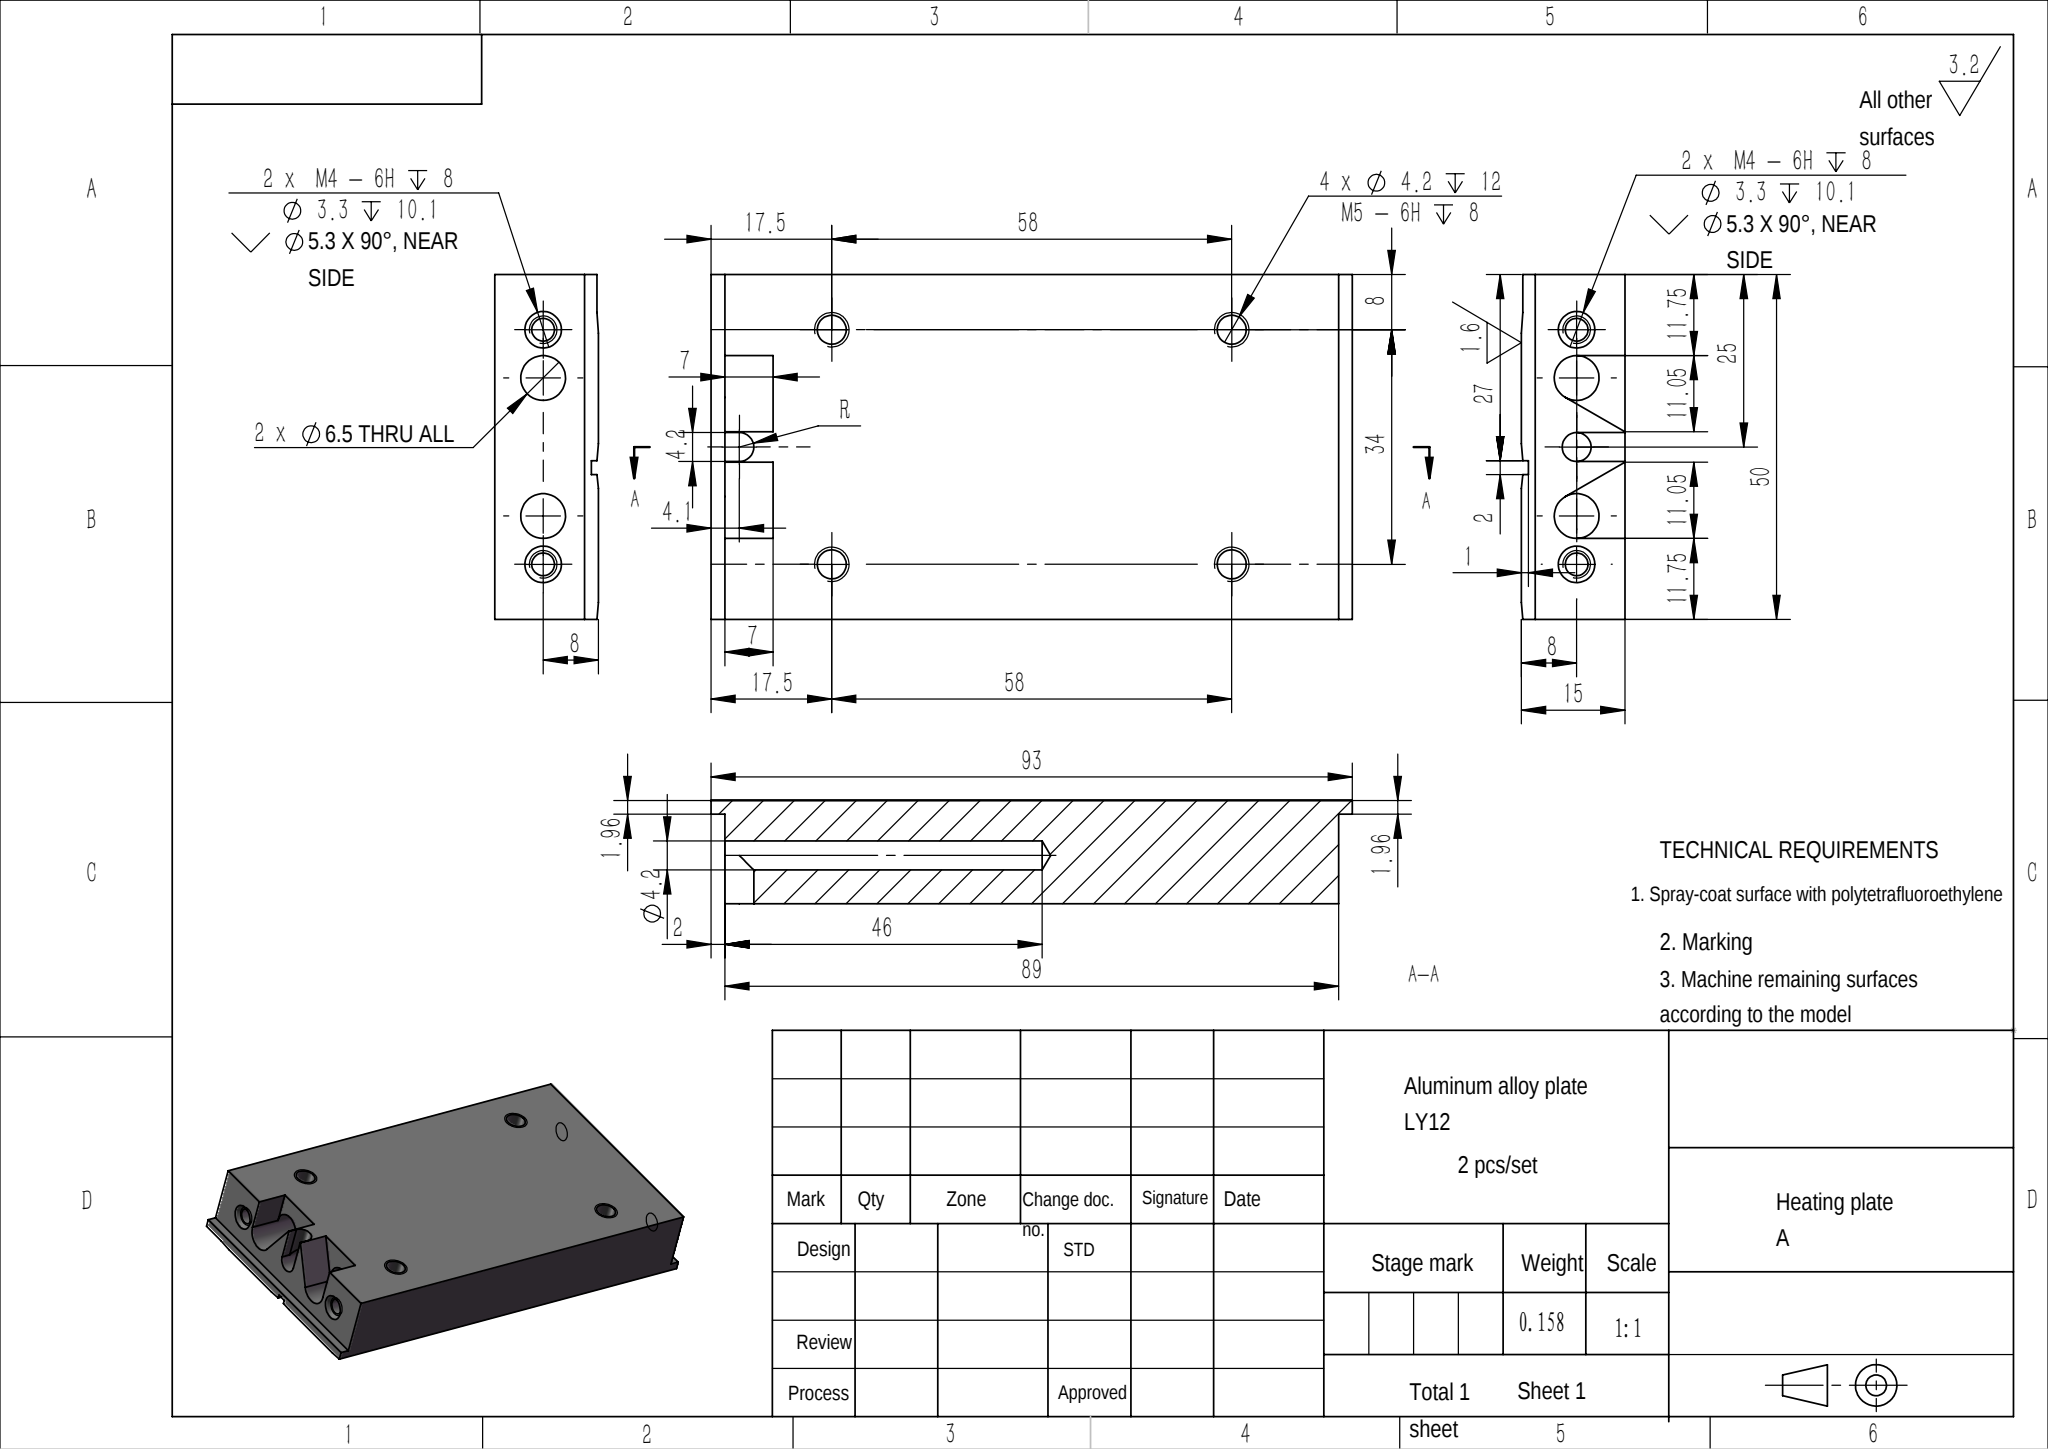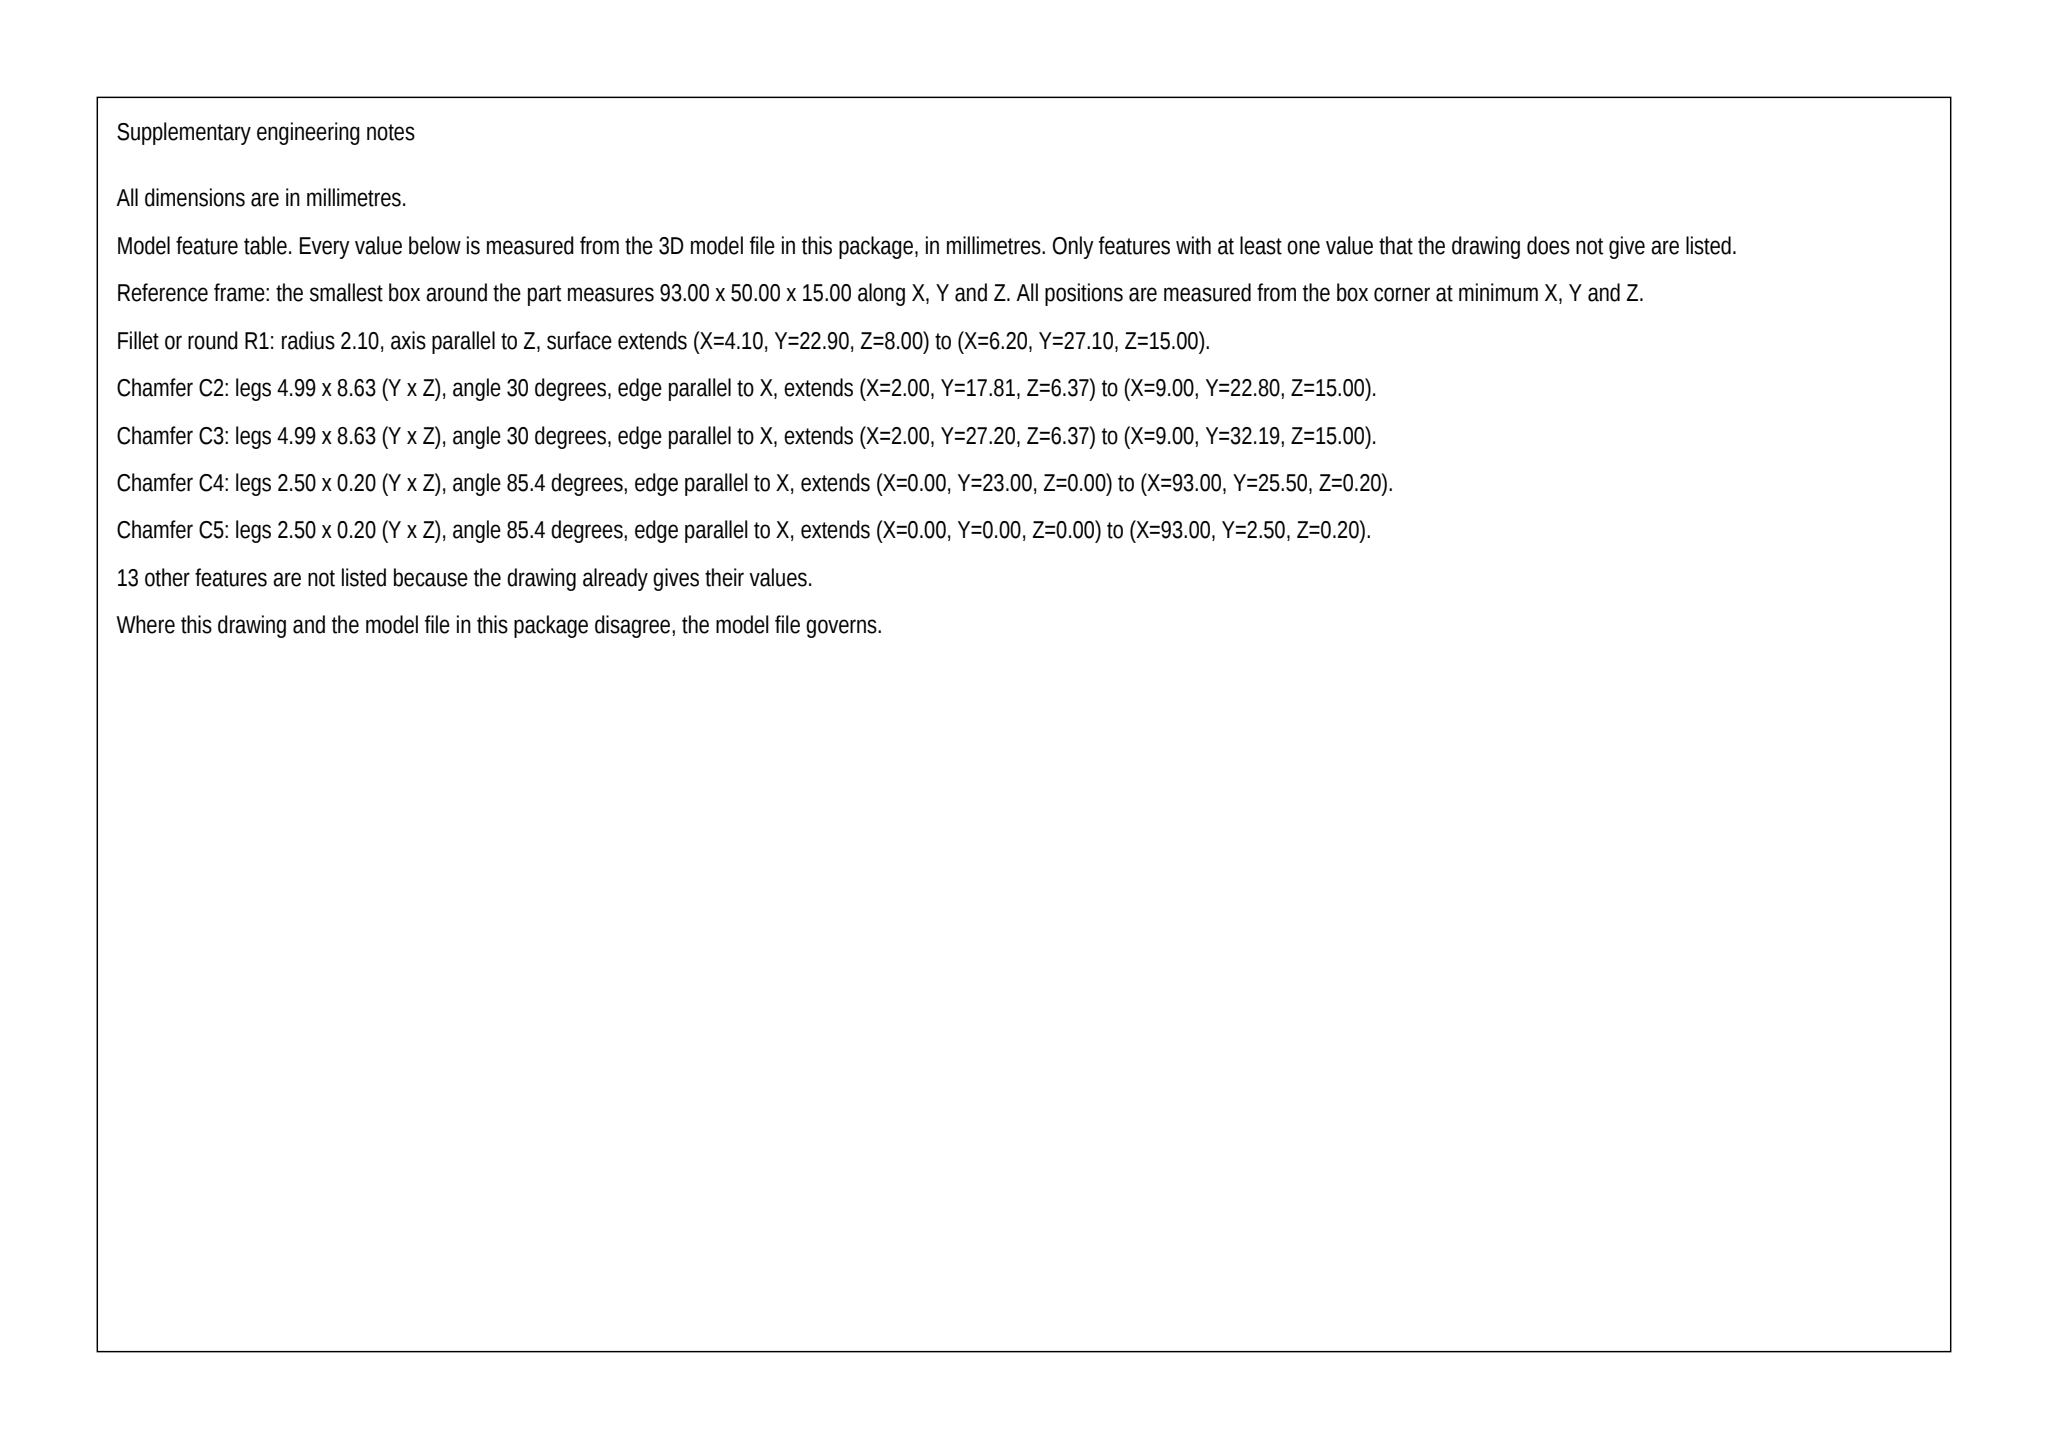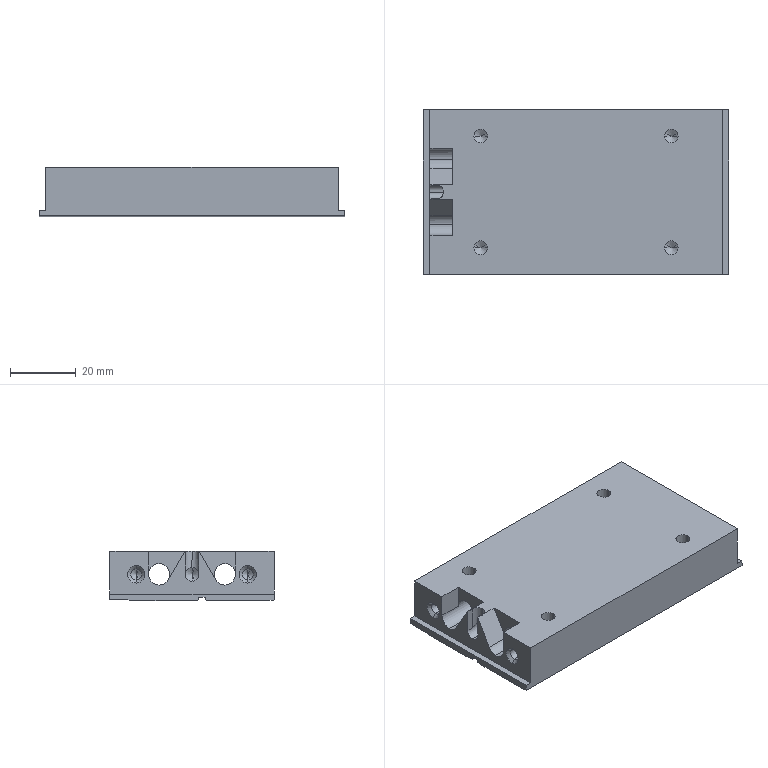Part | SolidWorks | mm | material Aluminum alloy plate LY12 | 1 solid | 77 faces | box 93 x 50 x 15 mm | volume 58409 mm3 | plane 27 | cone 26 | cylinder 24 | commonest cylinder face diameters 4.2 x12 3.3 x8 6.5 x4
build123d program:
from build123d import *

# Parameters (mm, degrees)
SKETCH1_W                      = 93
SKETCH1_H                      = 50
BOSS_EXTRUDE1_DEPTH            = 15
SKETCH2_W                      = 13.775
SKETCH2_H                      = 59.635
SKETCH2_W_2                    = 21.67
SKETCH2_H_2                    = 65.682
CUT_EXTRUDE1_DEPTH             = 13
F_6_5_6_5_DIAMETER_HOLE1_D     = 6.5
M4_TAPPED_HOLE1_D              = 3.3
M4_TAPPED_HOLE1_DEPTH          = 10.1
M4_TAPPED_HOLE1_CSINK_D        = 5.3
M4_TAPPED_HOLE1_CSINK_ANGLE    = 90
M4_TAPPED_HOLE1_TIP            = 0.9914
F_4_2_4_2_DIAMETER_HOLE1_D     = 4.2
F_4_2_4_2_DIAMETER_HOLE1_DEPTH = 46
F_4_2_4_2_DIAMETER_HOLE1_TIP   = 1.262
M4_TAPPED_HOLE2_D              = 3.3
M4_TAPPED_HOLE2_DEPTH          = 10.1
M4_TAPPED_HOLE2_CSINK_D        = 5.3
M4_TAPPED_HOLE2_CSINK_ANGLE    = 90
M4_TAPPED_HOLE2_TIP            = 0.9914
CUT_EXTRUDE3_REACH             = 56.884
CUT_EXTRUDE3_END_RADIUS        = 2.1
CUT_EXTRUDE4_START             = -7
CUT_EXTRUDE4_DEPTH             = 7
SKETCH17_W                     = 5.449
SKETCH17_H                     = 2
CUT_EXTRUDE5_DEPTH             = 98.463
M5_TAPPED_HOLE1_D              = 4.2
M5_TAPPED_HOLE1_DEPTH          = 12
M5_TAPPED_HOLE1_TIP            = 1.262
CUT_EXTRUDE6_DEPTH             = 98.463


with BuildPart() as part:
    # Sketch1 → Boss-Extrude1 (new body)
    with BuildSketch(Plane.XY):
        Rectangle(SKETCH1_W, SKETCH1_H)
    extrude(amount=-BOSS_EXTRUDE1_DEPTH)

    # Sketch2 → Cut-Extrude1 (cut)
    with BuildSketch(Plane.XY):
        with Locations((-51.387, 0.6719)):
            Rectangle(SKETCH2_W, SKETCH2_H)
        with Locations((55.335, -0.504)):
            Rectangle(SKETCH2_W_2, SKETCH2_H_2)
    extrude(amount=-CUT_EXTRUDE1_DEPTH, mode=Mode.SUBTRACT)

    # 6.5 _6.5_ Diameter Hole1 (through all)
    with Locations(Plane.ZY.offset(44.5)):
        with Locations((-7, 10), (-7, -10)):
            Hole(F_6_5_6_5_DIAMETER_HOLE1_D / 2)

    # M4 Tapped Hole1
    with Locations(Plane.ZY.offset(44.5)):
        with Locations((-7, 17), (-7, -17)):
            CounterSinkHole(M4_TAPPED_HOLE1_D / 2, M4_TAPPED_HOLE1_CSINK_D / 2, depth=M4_TAPPED_HOLE1_DEPTH, counter_sink_angle=M4_TAPPED_HOLE1_CSINK_ANGLE)
            with Locations((0, 0, -(M4_TAPPED_HOLE1_DEPTH + M4_TAPPED_HOLE1_TIP / 2))):  # 118° drill point
                Cone(0, M4_TAPPED_HOLE1_D / 2, M4_TAPPED_HOLE1_TIP, mode=Mode.SUBTRACT)

    # 4.2 _4.2_ Diameter Hole1
    with Locations(Plane.ZY.offset(44.5)):
        with Locations((-7, 0)):
            Hole(F_4_2_4_2_DIAMETER_HOLE1_D / 2, depth=F_4_2_4_2_DIAMETER_HOLE1_DEPTH)
            with Locations((0, 0, -(F_4_2_4_2_DIAMETER_HOLE1_DEPTH + F_4_2_4_2_DIAMETER_HOLE1_TIP / 2))):  # 118° drill point
                Cone(0, F_4_2_4_2_DIAMETER_HOLE1_D / 2, F_4_2_4_2_DIAMETER_HOLE1_TIP, mode=Mode.SUBTRACT)

    # M4 Tapped Hole2
    with Locations(Plane(origin=(44.5, 0, 0), x_dir=(0, 0, -1), z_dir=(1, 0, 0))):
        with Locations((7, 17), (7, -17)):
            CounterSinkHole(M4_TAPPED_HOLE2_D / 2, M4_TAPPED_HOLE2_CSINK_D / 2, depth=M4_TAPPED_HOLE2_DEPTH, counter_sink_angle=M4_TAPPED_HOLE2_CSINK_ANGLE)
            with Locations((0, 0, -(M4_TAPPED_HOLE2_DEPTH + M4_TAPPED_HOLE2_TIP / 2))):  # 118° drill point
                Cone(0, M4_TAPPED_HOLE2_D / 2, M4_TAPPED_HOLE2_TIP, mode=Mode.SUBTRACT)

    # Cut-Extrude3: up to this cylinder (the profile starts outside it)
    cut_extrude3_end = Plane(origin=(-42.596, 0, -7), z_dir=(-1, 0, 0)) * Cylinder(CUT_EXTRUDE3_END_RADIUS, 118.968, mode=Mode.PRIVATE)
    # Sketch15 → Cut-Extrude3 (cut, up to the surface)
    with BuildSketch(Plane.XY, mode=Mode.PRIVATE) as cut_extrude3_sk1:
        with BuildLine():
            Line((-42.4, 2.1), (-44.5, 2.1))
            Line((-44.5, 2.1), (-44.5, -2.1))
            Line((-44.5, -2.1), (-42.4, -2.1))
            ThreePointArc((-42.4, -2.1), (-40.3, 0), (-42.4, 2.1))
        make_face()
    cut_extrude3_tool1 = extrude(cut_extrude3_sk1.sketch, amount=-CUT_EXTRUDE3_REACH, mode=Mode.PRIVATE) - cut_extrude3_end
    add(cut_extrude3_tool1.solids().sort_by_distance((-42.596, 0, 0))[0], mode=Mode.SUBTRACT)

    # Sketch16 → Cut-Extrude4 (cut)
    with BuildSketch(Plane.ZY.offset(44.5).offset(CUT_EXTRUDE4_START)):
        with BuildLine():
            Line((0, -13.25), (0, -2.2))
            Line((0, -2.2), (-8.626, -7.186))
            ThreePointArc((-8.626, -7.186), (-10.139, -10.842), (-7, -13.25))
            Line((-7, -13.25), (0, -13.25))
        make_face()
        with BuildLine():
            Line((0, 13.25), (0, 2.2))
            Line((0, 2.2), (-8.626, 7.186))
            ThreePointArc((-8.626, 7.186), (-10.139, 10.842), (-7, 13.25))
            Line((-7, 13.25), (0, 13.25))
        make_face()
    extrude(amount=CUT_EXTRUDE4_DEPTH, mode=Mode.SUBTRACT)

    # Sketch17 → Cut-Extrude5 (cut, through all)
    with BuildSketch(Plane.ZY.offset(46.5)):
        with Locations((-16.724, -3)):
            Rectangle(SKETCH17_W, SKETCH17_H)
    extrude(amount=-CUT_EXTRUDE5_DEPTH, mode=Mode.SUBTRACT)

    # M5 Tapped Hole1
    with Locations(Plane.XY):
        with Locations((-29, 17), (29, 17), (-29, -17), (29, -17)):
            Hole(M5_TAPPED_HOLE1_D / 2, depth=M5_TAPPED_HOLE1_DEPTH)
            with Locations((0, 0, -(M5_TAPPED_HOLE1_DEPTH + M5_TAPPED_HOLE1_TIP / 2))):  # 118° drill point
                Cone(0, M5_TAPPED_HOLE1_D / 2, M5_TAPPED_HOLE1_TIP, mode=Mode.SUBTRACT)

    # Sketch20 → Cut-Extrude6 (cut, through all)
    with BuildSketch(Plane(origin=(46.5, 0, 0), x_dir=(0, 0, -1), z_dir=(1, 0, 0))):
        Polygon((14.8, 25), (14.8, 19.5), (15, 16.5), (15, 25), align=None)
        Polygon((15, 0.5), (14.8, -2), (15, -2), align=None)
        Polygon((14.8, -4), (15, -6), (15, -4), align=None)
        Polygon((15, -22.5), (14.8, -25), (15, -25), align=None)
    extrude(amount=-CUT_EXTRUDE6_DEPTH, mode=Mode.SUBTRACT)


solid = part.part